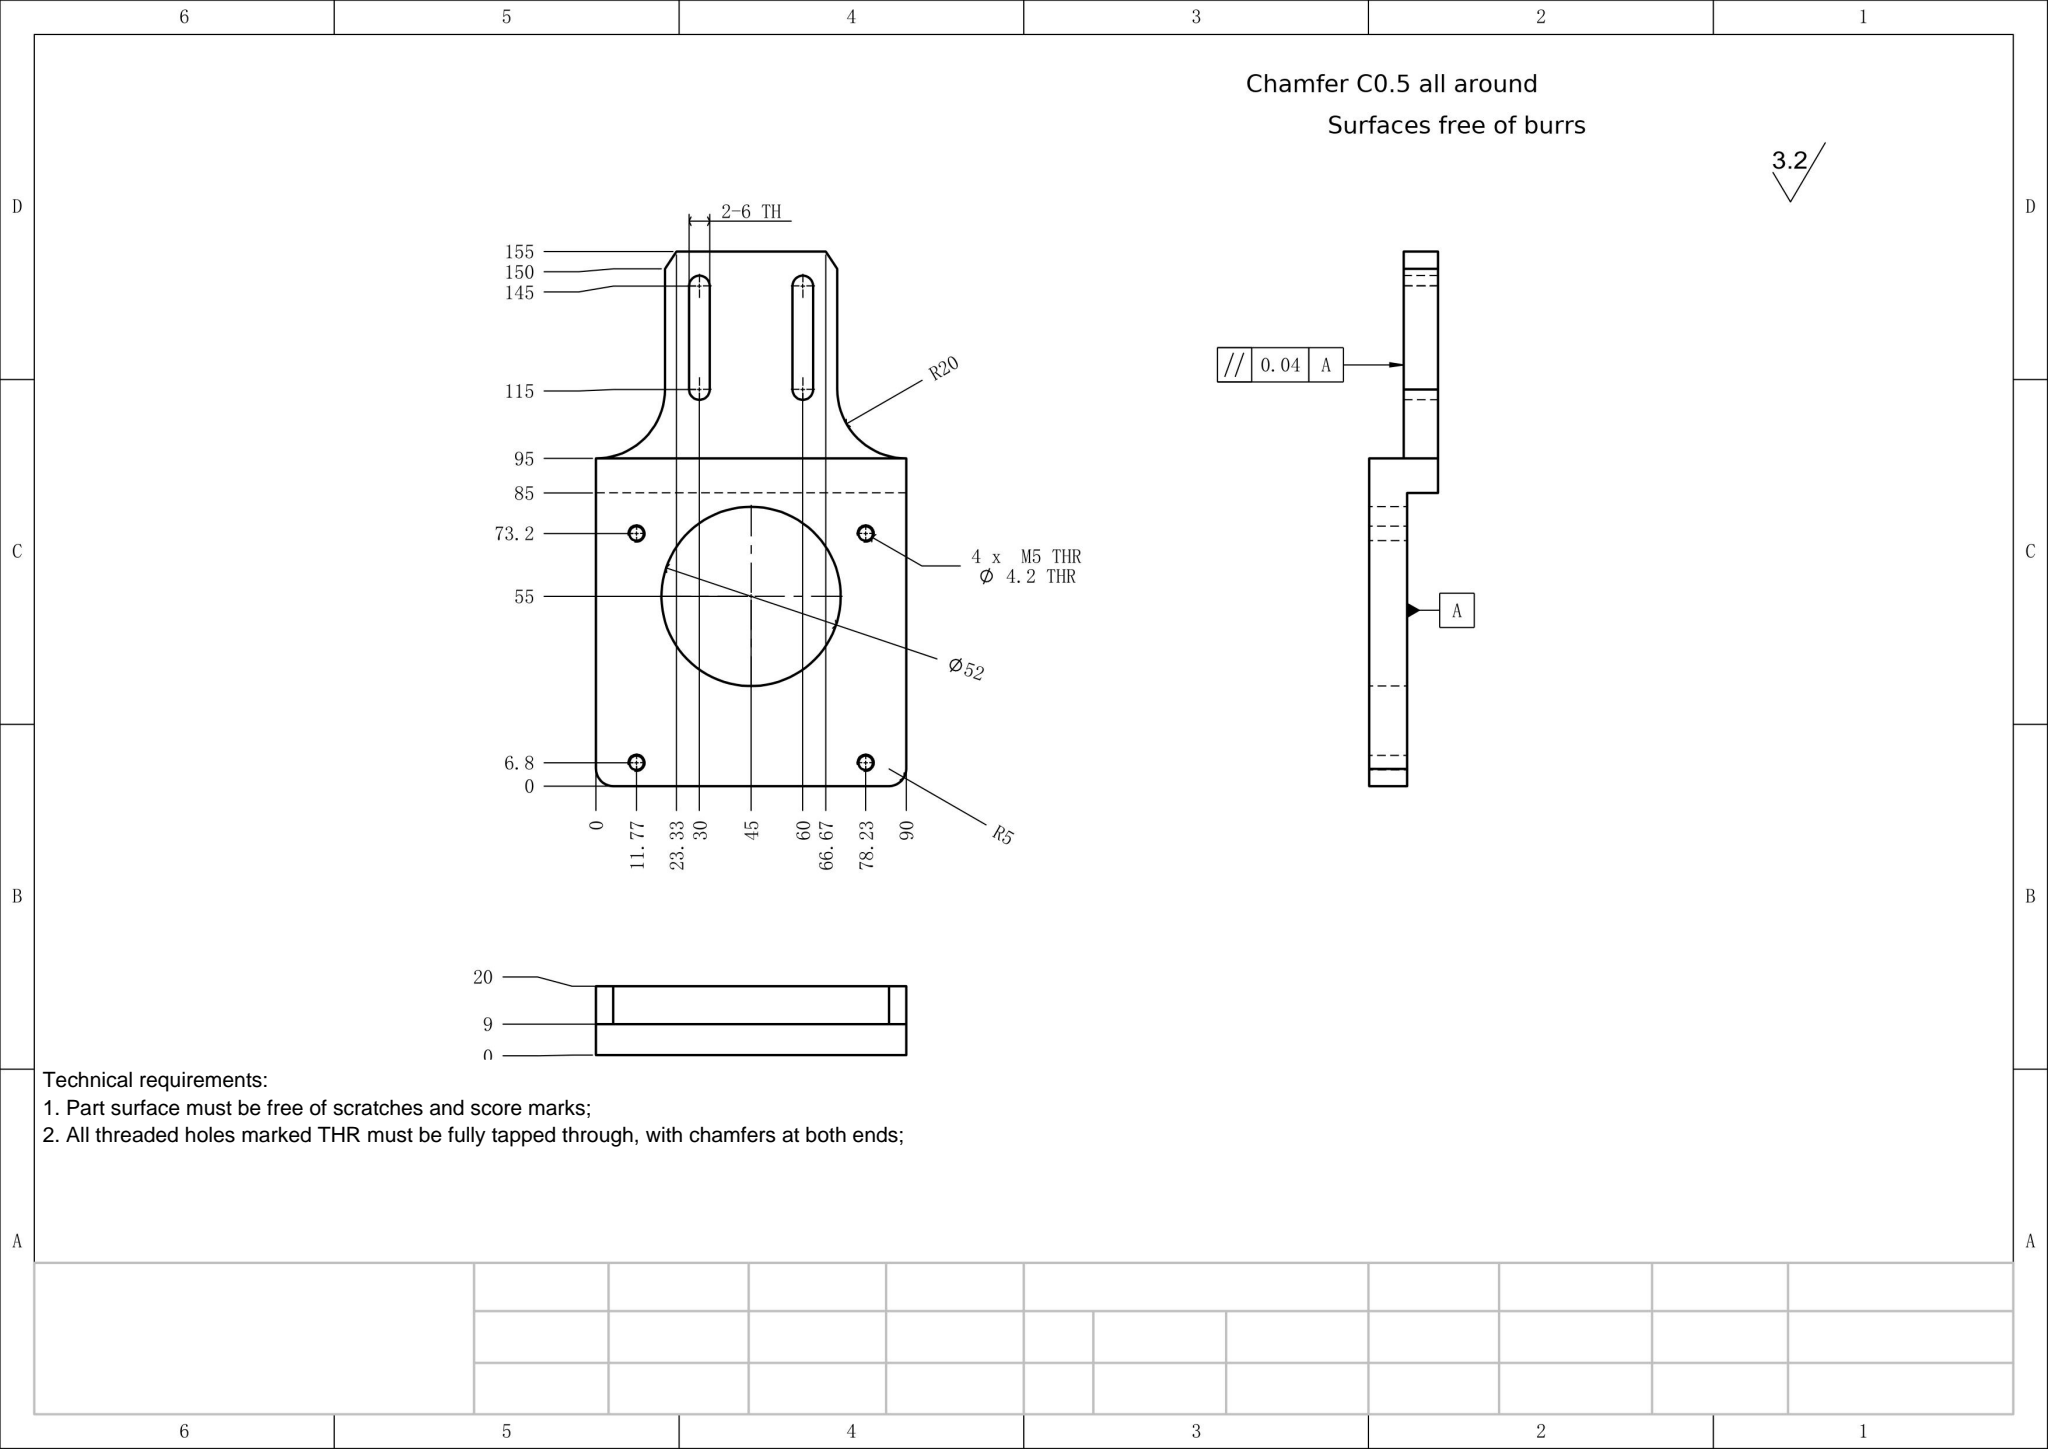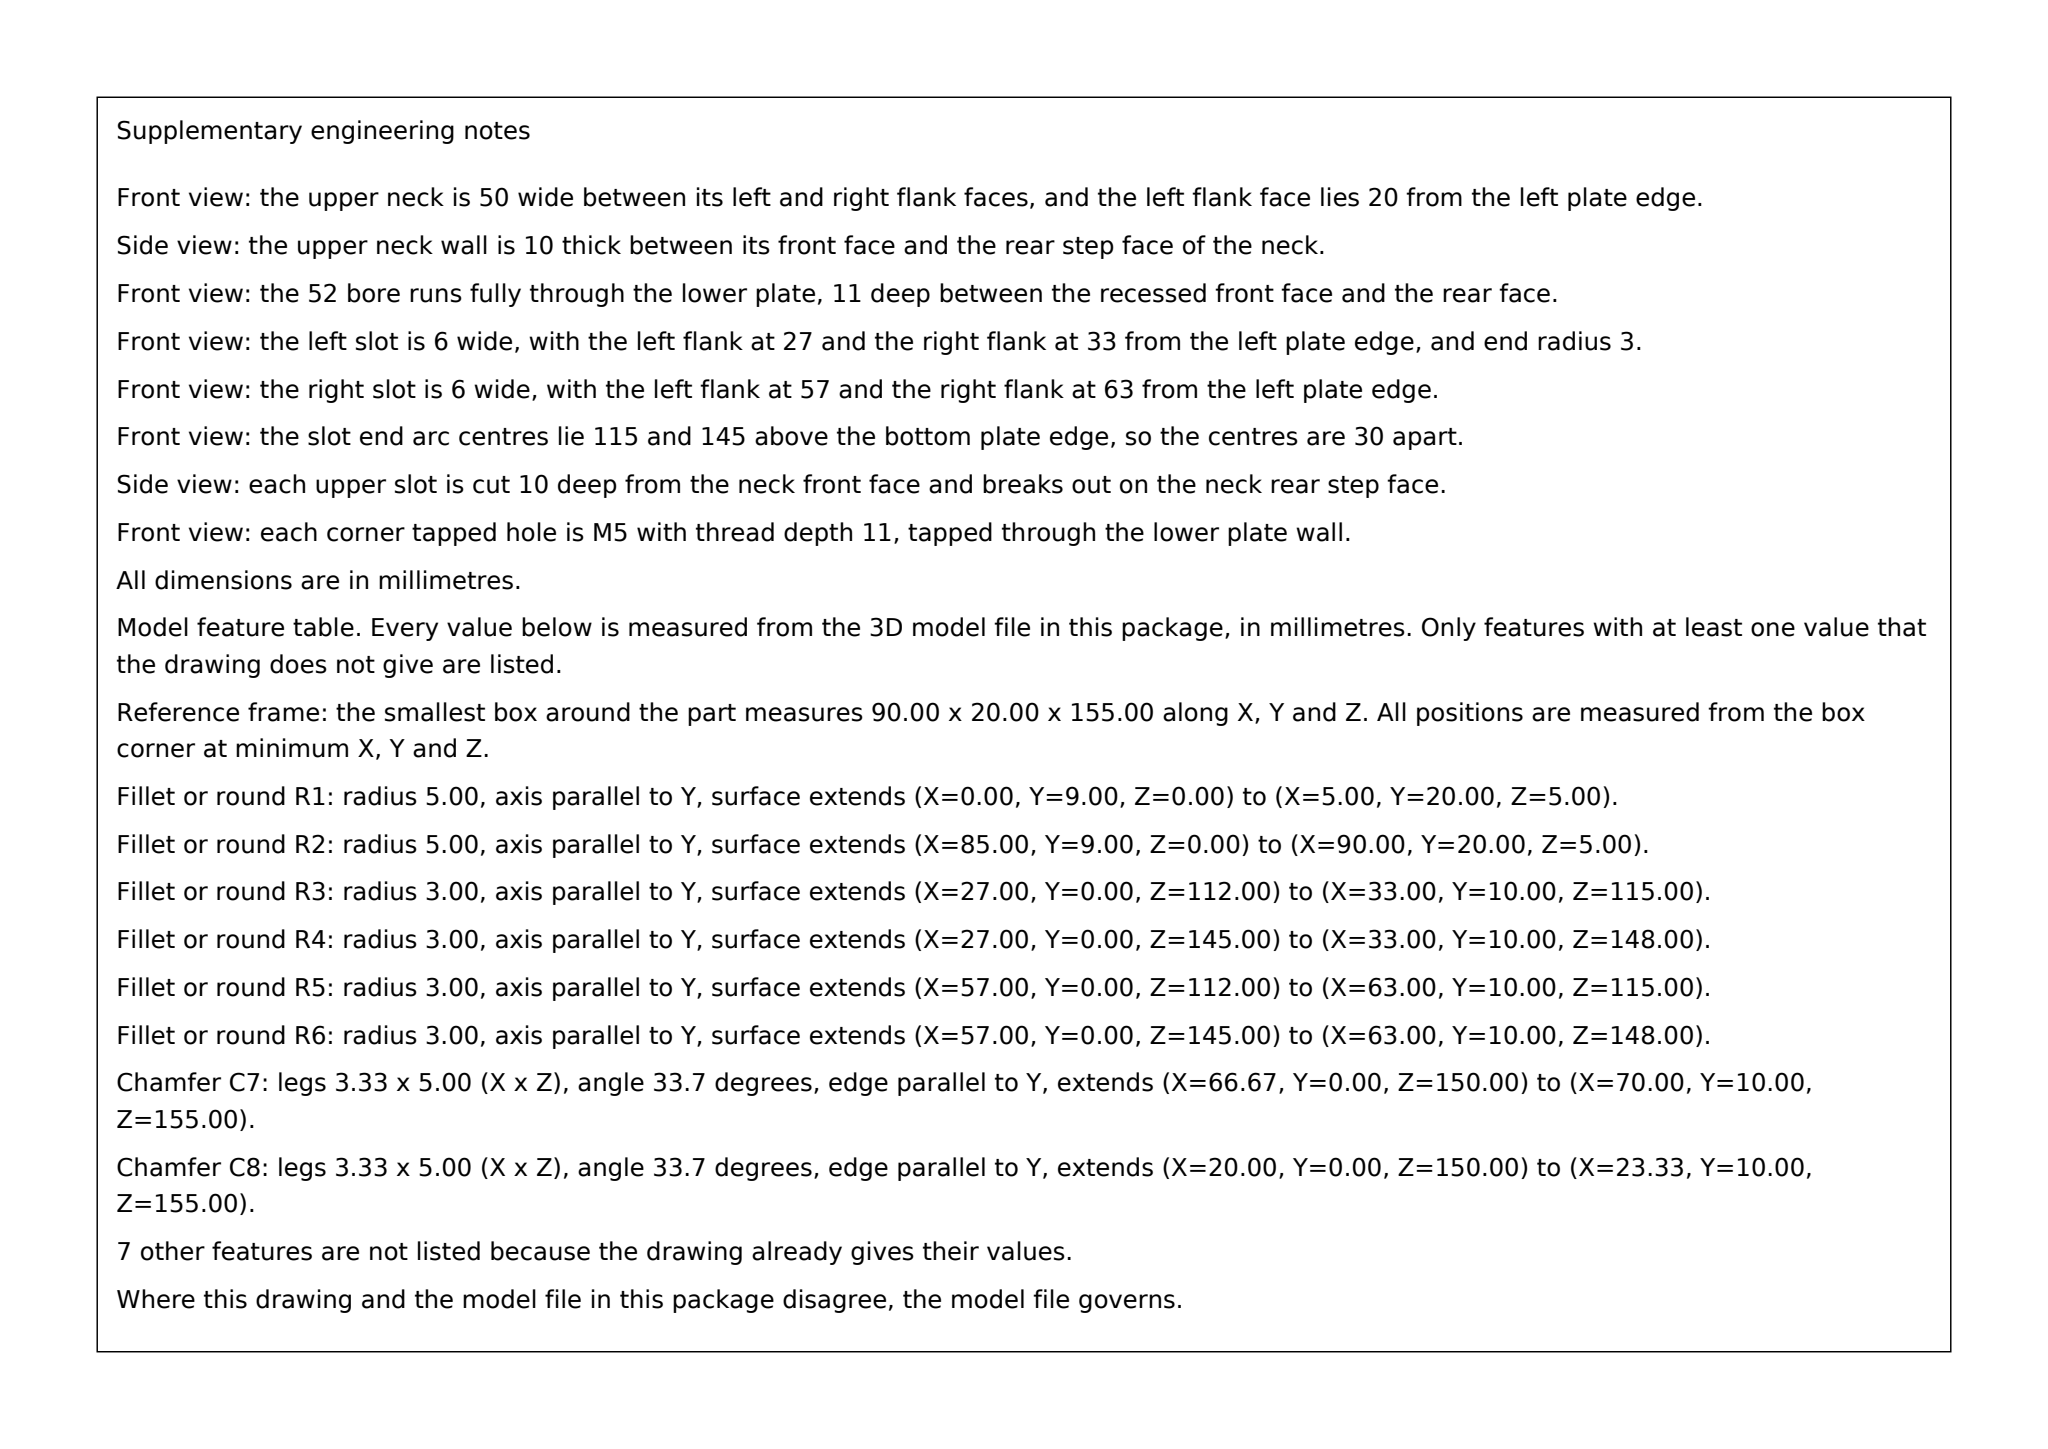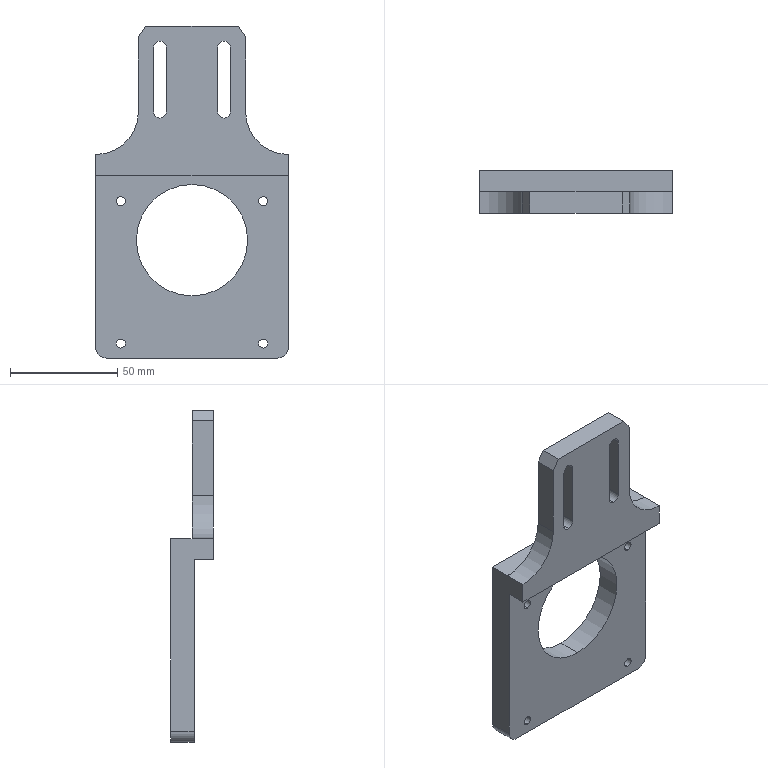Part | SolidWorks | mm | 1 solid | 38 faces | box 90 x 20 x 155 mm | volume 105446 mm3 | cylinder 20 | plane 18 | commonest cylinder face diameters 4.2 x8 6 x6 52 x2 10 x2 40 x2
Drawing notes:
Ø52 BORE THRU 11 THK PLATE | from the solid: cyl dia 52 axis y at (45,55), length 11 = plate thk (y planes 9 to 20)
UPPER BOSS 10 THK, FLUSH W/ BACK FACE | from the solid: boss spans y 10 to 20 = 10 thk; back face y=20 shared with plate